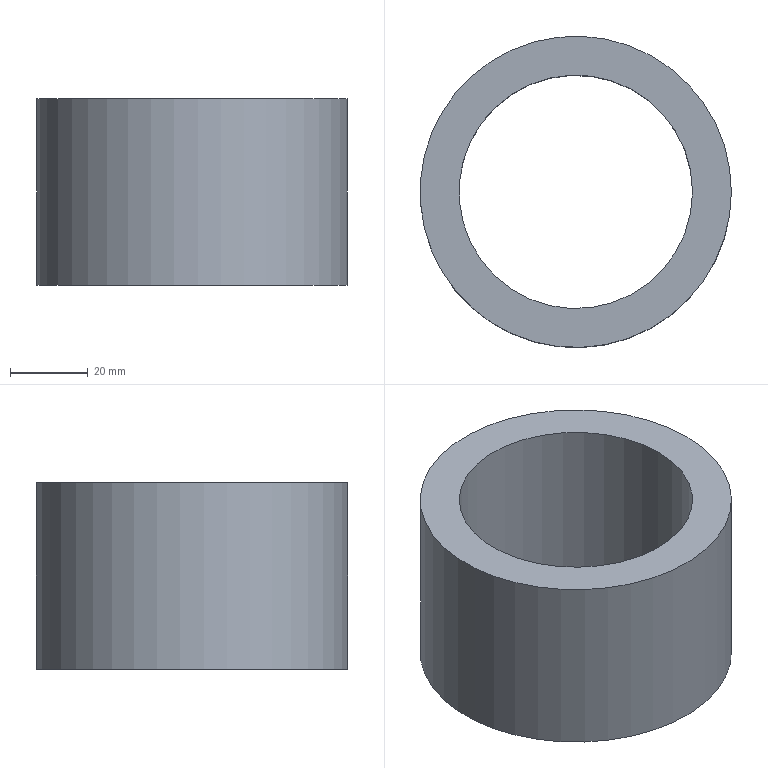Component | NX | CH3404_10-4 | 1 solid | 4 faces | box 80 x 80 x 48 mm | volume 105558 mm3 | cylinder 2 | plane 2 | commonest cylinder face diameters 80 x1 60 x1
STEP:
#1=CARTESIAN_POINT('',(0.,0.,0.));
#2=DIRECTION('',(0.,0.,1.));
#3=DIRECTION('',(1.,0.,0.));
#4=AXIS2_PLACEMENT_3D('',#1,#2,#3);
#5=CARTESIAN_POINT('',(40.,0.,130.));
#6=VERTEX_POINT('',#5);
#7=CARTESIAN_POINT('',(0.,0.,130.));
#8=DIRECTION('',(0.,0.,-1.));
#9=DIRECTION('',(1.,0.,0.));
#10=AXIS2_PLACEMENT_3D('',#7,#8,#9);
#11=CIRCLE('',#10,40.);
#12=CARTESIAN_POINT('',(0.,0.,130.));
#13=DIRECTION('',(0.,0.,-1.));
#14=DIRECTION('',(-1.,0.,0.));
#15=AXIS2_PLACEMENT_3D('',#12,#13,#14);
#16=CYLINDRICAL_SURFACE('',#15,40.);
#17=CARTESIAN_POINT('',(3.142,0.));
#18=DIRECTION('',(1.,0.));
#19=VECTOR('',#18,1.);
#20=LINE('',#17,#19);
#21=(GEOMETRIC_REPRESENTATION_CONTEXT(2)PARAMETRIC_REPRESENTATION_CONTEXT()REPRESENTATION_CONTEXT('',''));
#22=DEFINITIONAL_REPRESENTATION('',(#20),#21);
#23=PCURVE('',#16,#22);
#24=CARTESIAN_POINT('',(0.,0.,130.));
#25=DIRECTION('',(0.,0.,-1.));
#26=DIRECTION('',(-1.,0.,0.));
#27=AXIS2_PLACEMENT_3D('',#24,#25,#26);
#28=PLANE('',#27);
#29=CARTESIAN_POINT('',(0.,0.));
#30=DIRECTION('',(-1.,0.));
#31=AXIS2_PLACEMENT_2D('',#29,#30);
#32=CIRCLE('',#31,40.);
#33=(GEOMETRIC_REPRESENTATION_CONTEXT(2)PARAMETRIC_REPRESENTATION_CONTEXT()REPRESENTATION_CONTEXT('',''));
#34=DEFINITIONAL_REPRESENTATION('',(#32),#33);
#35=PCURVE('',#28,#34);
#36=SURFACE_CURVE('',#11,(#23,#35),.PCURVE_S1.);
#37=EDGE_CURVE('',#6,#6,#36,.T.);
#38=ORIENTED_EDGE('',*,*,#37,.T.);
#39=CARTESIAN_POINT('',(40.,0.,82.));
#40=VERTEX_POINT('',#39);
#41=CARTESIAN_POINT('',(40.,0.,130.));
#42=CARTESIAN_POINT('',(40.,0.,82.));
#43=B_SPLINE_CURVE_WITH_KNOTS('',1,(#41,#42),.UNSPECIFIED.,.F.,.F.,(2,2),(0.,48.),.PIECEWISE_BEZIER_KNOTS.);
#44=CARTESIAN_POINT('',(9.425,0.));
#45=DIRECTION('',(0.,1.));
#46=VECTOR('',#45,1.);
#47=LINE('',#44,#46);
#48=(GEOMETRIC_REPRESENTATION_CONTEXT(2)PARAMETRIC_REPRESENTATION_CONTEXT()REPRESENTATION_CONTEXT('',''));
#49=DEFINITIONAL_REPRESENTATION('',(#47),#48);
#50=PCURVE('',#16,#49);
#51=CARTESIAN_POINT('',(3.142,0.));
#52=DIRECTION('',(0.,1.));
#53=VECTOR('',#52,1.);
#54=LINE('',#51,#53);
#55=(GEOMETRIC_REPRESENTATION_CONTEXT(2)PARAMETRIC_REPRESENTATION_CONTEXT()REPRESENTATION_CONTEXT('',''));
#56=DEFINITIONAL_REPRESENTATION('',(#54),#55);
#57=PCURVE('',#16,#56);
#58=SEAM_CURVE('',#43,(#50,#57),.PCURVE_S1.);
#59=EDGE_CURVE('',#6,#40,#58,.T.);
#60=ORIENTED_EDGE('',*,*,#59,.T.);
#61=CARTESIAN_POINT('',(0.,0.,82.));
#62=DIRECTION('',(0.,0.,-1.));
#63=DIRECTION('',(1.,0.,0.));
#64=AXIS2_PLACEMENT_3D('',#61,#62,#63);
#65=CIRCLE('',#64,40.);
#66=CARTESIAN_POINT('',(3.142,48.));
#67=DIRECTION('',(1.,0.));
#68=VECTOR('',#67,1.);
#69=LINE('',#66,#68);
#70=(GEOMETRIC_REPRESENTATION_CONTEXT(2)PARAMETRIC_REPRESENTATION_CONTEXT()REPRESENTATION_CONTEXT('',''));
#71=DEFINITIONAL_REPRESENTATION('',(#69),#70);
#72=PCURVE('',#16,#71);
#73=CARTESIAN_POINT('',(0.,0.,82.));
#74=DIRECTION('',(0.,0.,-1.));
#75=DIRECTION('',(-1.,0.,0.));
#76=AXIS2_PLACEMENT_3D('',#73,#74,#75);
#77=PLANE('',#76);
#78=CARTESIAN_POINT('',(0.,0.));
#79=DIRECTION('',(-1.,0.));
#80=AXIS2_PLACEMENT_2D('',#78,#79);
#81=CIRCLE('',#80,40.);
#82=(GEOMETRIC_REPRESENTATION_CONTEXT(2)PARAMETRIC_REPRESENTATION_CONTEXT()REPRESENTATION_CONTEXT('',''));
#83=DEFINITIONAL_REPRESENTATION('',(#81),#82);
#84=PCURVE('',#77,#83);
#85=SURFACE_CURVE('',#65,(#72,#84),.PCURVE_S1.);
#86=EDGE_CURVE('',#40,#40,#85,.T.);
#87=ORIENTED_EDGE('',*,*,#86,.F.);
#88=ORIENTED_EDGE('',*,*,#59,.F.);
#89=EDGE_LOOP('',(#38,#60,#87,#88));
#90=FACE_BOUND('',#89,.T.);
#91=ADVANCED_FACE('',(#90),#16,.T.);
#92=CARTESIAN_POINT('',(30.,0.,130.));
#93=VERTEX_POINT('',#92);
#94=CARTESIAN_POINT('',(0.,0.,130.));
#95=DIRECTION('',(0.,0.,-1.));
#96=DIRECTION('',(1.,0.,0.));
#97=AXIS2_PLACEMENT_3D('',#94,#95,#96);
#98=CIRCLE('',#97,30.);
#99=CARTESIAN_POINT('',(0.,0.,130.));
#100=DIRECTION('',(0.,0.,-1.));
#101=DIRECTION('',(-1.,0.,0.));
#102=AXIS2_PLACEMENT_3D('',#99,#100,#101);
#103=CYLINDRICAL_SURFACE('',#102,30.);
#104=CARTESIAN_POINT('',(3.142,0.));
#105=DIRECTION('',(1.,0.));
#106=VECTOR('',#105,1.);
#107=LINE('',#104,#106);
#108=(GEOMETRIC_REPRESENTATION_CONTEXT(2)PARAMETRIC_REPRESENTATION_CONTEXT()REPRESENTATION_CONTEXT('',''));
#109=DEFINITIONAL_REPRESENTATION('',(#107),#108);
#110=PCURVE('',#103,#109);
#111=CARTESIAN_POINT('',(0.,0.));
#112=DIRECTION('',(-1.,0.));
#113=AXIS2_PLACEMENT_2D('',#111,#112);
#114=CIRCLE('',#113,30.);
#115=(GEOMETRIC_REPRESENTATION_CONTEXT(2)PARAMETRIC_REPRESENTATION_CONTEXT()REPRESENTATION_CONTEXT('',''));
#116=DEFINITIONAL_REPRESENTATION('',(#114),#115);
#117=PCURVE('',#28,#116);
#118=SURFACE_CURVE('',#98,(#110,#117),.PCURVE_S1.);
#119=EDGE_CURVE('',#93,#93,#118,.T.);
#120=ORIENTED_EDGE('',*,*,#119,.T.);
#121=CARTESIAN_POINT('',(30.,0.,82.));
#122=VERTEX_POINT('',#121);
#123=CARTESIAN_POINT('',(30.,0.,130.));
#124=CARTESIAN_POINT('',(30.,0.,82.));
#125=B_SPLINE_CURVE_WITH_KNOTS('',1,(#123,#124),.UNSPECIFIED.,.F.,.F.,(2,2),(0.,48.),.PIECEWISE_BEZIER_KNOTS.);
#126=CARTESIAN_POINT('',(9.425,0.));
#127=DIRECTION('',(0.,1.));
#128=VECTOR('',#127,1.);
#129=LINE('',#126,#128);
#130=(GEOMETRIC_REPRESENTATION_CONTEXT(2)PARAMETRIC_REPRESENTATION_CONTEXT()REPRESENTATION_CONTEXT('',''));
#131=DEFINITIONAL_REPRESENTATION('',(#129),#130);
#132=PCURVE('',#103,#131);
#133=CARTESIAN_POINT('',(3.142,0.));
#134=DIRECTION('',(0.,1.));
#135=VECTOR('',#134,1.);
#136=LINE('',#133,#135);
#137=(GEOMETRIC_REPRESENTATION_CONTEXT(2)PARAMETRIC_REPRESENTATION_CONTEXT()REPRESENTATION_CONTEXT('',''));
#138=DEFINITIONAL_REPRESENTATION('',(#136),#137);
#139=PCURVE('',#103,#138);
#140=SEAM_CURVE('',#125,(#132,#139),.PCURVE_S1.);
#141=EDGE_CURVE('',#93,#122,#140,.T.);
#142=ORIENTED_EDGE('',*,*,#141,.T.);
#143=CARTESIAN_POINT('',(0.,0.,82.));
#144=DIRECTION('',(0.,0.,-1.));
#145=DIRECTION('',(1.,0.,0.));
#146=AXIS2_PLACEMENT_3D('',#143,#144,#145);
#147=CIRCLE('',#146,30.);
#148=CARTESIAN_POINT('',(3.142,48.));
#149=DIRECTION('',(1.,0.));
#150=VECTOR('',#149,1.);
#151=LINE('',#148,#150);
#152=(GEOMETRIC_REPRESENTATION_CONTEXT(2)PARAMETRIC_REPRESENTATION_CONTEXT()REPRESENTATION_CONTEXT('',''));
#153=DEFINITIONAL_REPRESENTATION('',(#151),#152);
#154=PCURVE('',#103,#153);
#155=CARTESIAN_POINT('',(0.,0.));
#156=DIRECTION('',(-1.,0.));
#157=AXIS2_PLACEMENT_2D('',#155,#156);
#158=CIRCLE('',#157,30.);
#159=(GEOMETRIC_REPRESENTATION_CONTEXT(2)PARAMETRIC_REPRESENTATION_CONTEXT()REPRESENTATION_CONTEXT('',''));
#160=DEFINITIONAL_REPRESENTATION('',(#158),#159);
#161=PCURVE('',#77,#160);
#162=SURFACE_CURVE('',#147,(#154,#161),.PCURVE_S1.);
#163=EDGE_CURVE('',#122,#122,#162,.T.);
#164=ORIENTED_EDGE('',*,*,#163,.F.);
#165=ORIENTED_EDGE('',*,*,#141,.F.);
#166=EDGE_LOOP('',(#120,#142,#164,#165));
#167=FACE_BOUND('',#166,.F.);
#168=ADVANCED_FACE('',(#167),#103,.F.);
#169=ORIENTED_EDGE('',*,*,#37,.F.);
#170=EDGE_LOOP('',(#169));
#171=FACE_BOUND('',#170,.T.);
#172=ORIENTED_EDGE('',*,*,#119,.T.);
#173=EDGE_LOOP('',(#172));
#174=FACE_BOUND('',#173,.T.);
#175=ADVANCED_FACE('',(#171,#174),#28,.F.);
#176=ORIENTED_EDGE('',*,*,#86,.T.);
#177=EDGE_LOOP('',(#176));
#178=FACE_BOUND('',#177,.T.);
#179=ORIENTED_EDGE('',*,*,#163,.F.);
#180=EDGE_LOOP('',(#179));
#181=FACE_BOUND('',#180,.T.);
#182=ADVANCED_FACE('',(#178,#181),#77,.T.);
#183=CLOSED_SHELL('',(#91,#168,#175,#182));
#184=MANIFOLD_SOLID_BREP('',#183);
#185=(LENGTH_UNIT()NAMED_UNIT(*)SI_UNIT(.MILLI.,.METRE.));
#186=UNCERTAINTY_MEASURE_WITH_UNIT(LENGTH_MEASURE(0.00001),#185,'','');
#187=(NAMED_UNIT(*)PLANE_ANGLE_UNIT()SI_UNIT($,.RADIAN.));
#188=(NAMED_UNIT(*)SI_UNIT($,.STERADIAN.)SOLID_ANGLE_UNIT());
#189=(GEOMETRIC_REPRESENTATION_CONTEXT(3)GLOBAL_UNCERTAINTY_ASSIGNED_CONTEXT((#186))GLOBAL_UNIT_ASSIGNED_CONTEXT((#185,#187,#188))REPRESENTATION_CONTEXT('',''));
#190=ADVANCED_BREP_SHAPE_REPRESENTATION('',(#4,#184),#189);